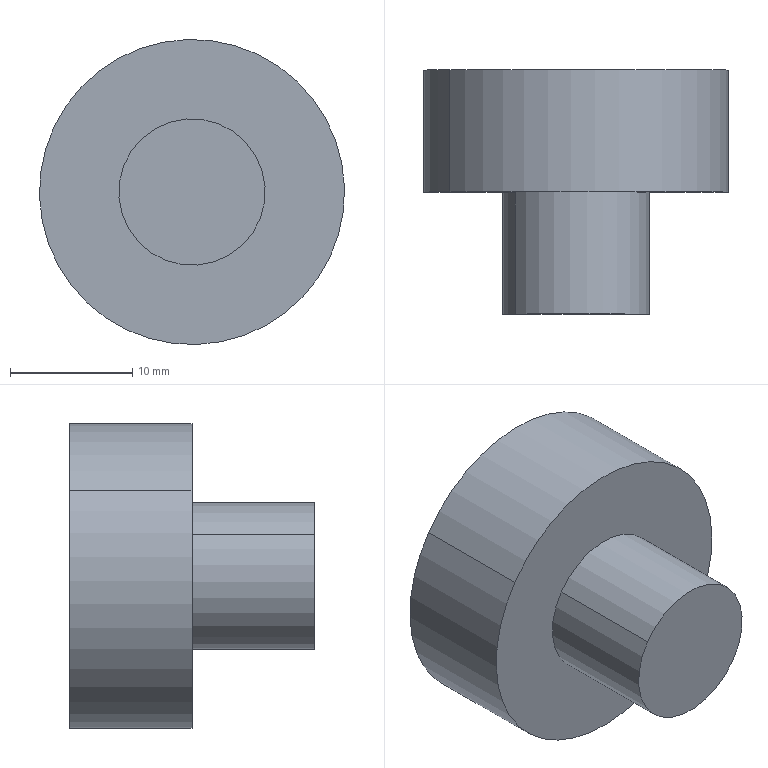Component | SolidWorks | UpperAxis-1_UpperSlideFixedBlock-1 | 1 solid | 10 faces | box 25 x 20 x 25 mm | volume 5870 mm3 | cylinder 6 | plane 4 | commonest cylinder face diameters 5.2 x2 12 x2 25 x2
build123d program:
from build123d import *

# Parameters (mm, degrees)
SKETCH1_R           = 12.5
BOSS_EXTRUDE1_DEPTH = 10
SKETCH2_R           = 6
BOSS_EXTRUDE2_DEPTH = 10
SKETCH3_R           = 2.6
CUT_EXTRUDE1_DEPTH  = 8


with BuildPart() as part:
    # Sketch1 → Boss-Extrude1 (new body)
    with BuildSketch(Plane.XY):
        Circle(SKETCH1_R)
    extrude(amount=BOSS_EXTRUDE1_DEPTH)

    # Sketch2 → Boss-Extrude2 (add)
    with BuildSketch(Plane.XY.offset(10)):
        Circle(SKETCH2_R)
    extrude(amount=BOSS_EXTRUDE2_DEPTH)

    # Sketch3 → Cut-Extrude1 (cut)
    with BuildSketch(Plane(origin=(0, 0, 0), x_dir=(-1, 0, 0), z_dir=(0, 0, -1))):
        Circle(SKETCH3_R)
    extrude(amount=-CUT_EXTRUDE1_DEPTH, mode=Mode.SUBTRACT)


solid = part.part

# Placed as in the assembly
solid = solid.moved(Location((-778.65, 394.568, -31.569), (90, 0, 0)))
STEP:
#1=COLOUR_RGB('',0.7922,0.8196,0.9333);
#2=FILL_AREA_STYLE_COLOUR('',#1);
#3=FILL_AREA_STYLE('',(#2));
#4=SURFACE_STYLE_FILL_AREA(#3);
#5=SURFACE_SIDE_STYLE('',(#4));
#6=SURFACE_STYLE_USAGE(.BOTH.,#5);
#7=PRESENTATION_STYLE_ASSIGNMENT((#6));
#8=CARTESIAN_POINT('',(-30.571,15.219,-1.301));
#9=VERTEX_POINT('',#8);
#10=CARTESIAN_POINT('',(-30.74,15.219,-1.185));
#11=VERTEX_POINT('',#10);
#12=CARTESIAN_POINT('',(-30.655,15.219,-1.243));
#13=DIRECTION('',(-0.,1.,0.));
#14=DIRECTION('',(-0.8265,0.,0.563));
#15=AXIS2_PLACEMENT_3D('',#12,#13,#14);
#16=CIRCLE('',#15,0.1024);
#17=EDGE_CURVE('',#9,#11,#16,.T.);
#18=ORIENTED_EDGE('',*,*,#17,.F.);
#19=CARTESIAN_POINT('',(-30.571,15.534,-1.301));
#20=VERTEX_POINT('',#19);
#21=CARTESIAN_POINT('',(-30.571,15.219,-1.301));
#22=DIRECTION('',(-0.,1.,0.));
#23=VECTOR('',#22,39.37);
#24=LINE('',#21,#23);
#25=EDGE_CURVE('',#9,#20,#24,.T.);
#26=ORIENTED_EDGE('',*,*,#25,.T.);
#27=CARTESIAN_POINT('',(-30.74,15.534,-1.185));
#28=VERTEX_POINT('',#27);
#29=CARTESIAN_POINT('',(-30.655,15.534,-1.243));
#30=DIRECTION('',(-0.,1.,0.));
#31=DIRECTION('',(-0.8265,0.,0.563));
#32=AXIS2_PLACEMENT_3D('',#29,#30,#31);
#33=CIRCLE('',#32,0.1024);
#34=EDGE_CURVE('',#20,#28,#33,.T.);
#35=ORIENTED_EDGE('',*,*,#34,.T.);
#36=CARTESIAN_POINT('',(-30.74,15.219,-1.185));
#37=DIRECTION('',(-0.,1.,0.));
#38=VECTOR('',#37,39.37);
#39=LINE('',#36,#38);
#40=EDGE_CURVE('',#11,#28,#39,.T.);
#41=ORIENTED_EDGE('',*,*,#40,.F.);
#42=EDGE_LOOP('',(#18,#26,#35,#41));
#43=FACE_OUTER_BOUND('',#42,.T.);
#44=CARTESIAN_POINT('',(-30.655,15.219,-1.243));
#45=DIRECTION('',(-0.,1.,0.));
#46=DIRECTION('',(-0.8265,0.,0.563));
#47=AXIS2_PLACEMENT_3D('',#44,#45,#46);
#48=CYLINDRICAL_SURFACE('',#47,0.1024);
#49=ADVANCED_FACE('',(#43),#48,.F.);
#50=CARTESIAN_POINT('',(-30.46,14.747,-1.376));
#51=VERTEX_POINT('',#50);
#52=CARTESIAN_POINT('',(-30.851,14.747,-1.11));
#53=VERTEX_POINT('',#52);
#54=CARTESIAN_POINT('',(-30.655,14.747,-1.243));
#55=DIRECTION('',(0.,-1.,-0.));
#56=DIRECTION('',(0.8265,0.,-0.563));
#57=AXIS2_PLACEMENT_3D('',#54,#55,#56);
#58=CIRCLE('',#57,0.2362);
#59=EDGE_CURVE('',#51,#53,#58,.T.);
#60=ORIENTED_EDGE('',*,*,#59,.F.);
#61=CARTESIAN_POINT('',(-30.46,15.14,-1.376));
#62=VERTEX_POINT('',#61);
#63=CARTESIAN_POINT('',(-30.46,14.747,-1.376));
#64=DIRECTION('',(-0.,1.,0.));
#65=VECTOR('',#64,39.37);
#66=LINE('',#63,#65);
#67=EDGE_CURVE('',#51,#62,#66,.T.);
#68=ORIENTED_EDGE('',*,*,#67,.T.);
#69=CARTESIAN_POINT('',(-30.851,15.14,-1.11));
#70=VERTEX_POINT('',#69);
#71=CARTESIAN_POINT('',(-30.655,15.14,-1.243));
#72=DIRECTION('',(0.,-1.,-0.));
#73=DIRECTION('',(0.8265,0.,-0.563));
#74=AXIS2_PLACEMENT_3D('',#71,#72,#73);
#75=CIRCLE('',#74,0.2362);
#76=EDGE_CURVE('',#62,#70,#75,.T.);
#77=ORIENTED_EDGE('',*,*,#76,.T.);
#78=CARTESIAN_POINT('',(-30.851,14.747,-1.11));
#79=DIRECTION('',(-0.,1.,0.));
#80=VECTOR('',#79,39.37);
#81=LINE('',#78,#80);
#82=EDGE_CURVE('',#53,#70,#81,.T.);
#83=ORIENTED_EDGE('',*,*,#82,.F.);
#84=EDGE_LOOP('',(#60,#68,#77,#83));
#85=FACE_OUTER_BOUND('',#84,.T.);
#86=CARTESIAN_POINT('',(-30.655,14.747,-1.243));
#87=DIRECTION('',(-0.,1.,0.));
#88=DIRECTION('',(-0.8265,0.,0.563));
#89=AXIS2_PLACEMENT_3D('',#86,#87,#88);
#90=CYLINDRICAL_SURFACE('',#89,0.2362);
#91=ADVANCED_FACE('',(#85),#90,.T.);
#92=CARTESIAN_POINT('',(-30.249,15.14,-1.52));
#93=VERTEX_POINT('',#92);
#94=CARTESIAN_POINT('',(-31.062,15.14,-0.9658));
#95=VERTEX_POINT('',#94);
#96=CARTESIAN_POINT('',(-30.655,15.14,-1.243));
#97=DIRECTION('',(0.,-1.,-0.));
#98=DIRECTION('',(0.8265,0.,-0.563));
#99=AXIS2_PLACEMENT_3D('',#96,#97,#98);
#100=CIRCLE('',#99,0.4921);
#101=EDGE_CURVE('',#93,#95,#100,.T.);
#102=ORIENTED_EDGE('',*,*,#101,.F.);
#103=CARTESIAN_POINT('',(-30.249,15.534,-1.52));
#104=VERTEX_POINT('',#103);
#105=CARTESIAN_POINT('',(-30.249,15.14,-1.52));
#106=DIRECTION('',(-0.,1.,0.));
#107=VECTOR('',#106,39.37);
#108=LINE('',#105,#107);
#109=EDGE_CURVE('',#93,#104,#108,.T.);
#110=ORIENTED_EDGE('',*,*,#109,.T.);
#111=CARTESIAN_POINT('',(-31.062,15.534,-0.9658));
#112=VERTEX_POINT('',#111);
#113=CARTESIAN_POINT('',(-30.655,15.534,-1.243));
#114=DIRECTION('',(0.,-1.,-0.));
#115=DIRECTION('',(0.8265,0.,-0.563));
#116=AXIS2_PLACEMENT_3D('',#113,#114,#115);
#117=CIRCLE('',#116,0.4921);
#118=EDGE_CURVE('',#104,#112,#117,.T.);
#119=ORIENTED_EDGE('',*,*,#118,.T.);
#120=CARTESIAN_POINT('',(-31.062,15.14,-0.9658));
#121=DIRECTION('',(-0.,1.,0.));
#122=VECTOR('',#121,39.37);
#123=LINE('',#120,#122);
#124=EDGE_CURVE('',#95,#112,#123,.T.);
#125=ORIENTED_EDGE('',*,*,#124,.F.);
#126=EDGE_LOOP('',(#102,#110,#119,#125));
#127=FACE_OUTER_BOUND('',#126,.T.);
#128=CARTESIAN_POINT('',(-30.655,15.14,-1.243));
#129=DIRECTION('',(-0.,1.,0.));
#130=DIRECTION('',(-0.8265,0.,0.563));
#131=AXIS2_PLACEMENT_3D('',#128,#129,#130);
#132=CYLINDRICAL_SURFACE('',#131,0.4921);
#133=ADVANCED_FACE('',(#127),#132,.T.);
#134=CARTESIAN_POINT('',(-30.655,15.14,-1.243));
#135=DIRECTION('',(0.,-1.,-0.));
#136=DIRECTION('',(0.8265,0.,-0.563));
#137=AXIS2_PLACEMENT_3D('',#134,#135,#136);
#138=CIRCLE('',#137,0.4921);
#139=EDGE_CURVE('',#95,#93,#138,.T.);
#140=ORIENTED_EDGE('',*,*,#139,.T.);
#141=ORIENTED_EDGE('',*,*,#101,.T.);
#142=EDGE_LOOP('',(#140,#141));
#143=FACE_OUTER_BOUND('',#142,.T.);
#144=CARTESIAN_POINT('',(-30.655,15.14,-1.243));
#145=DIRECTION('',(0.,-1.,-0.));
#146=DIRECTION('',(0.8265,0.,-0.563));
#147=AXIS2_PLACEMENT_3D('',#144,#145,#146);
#148=CIRCLE('',#147,0.2362);
#149=EDGE_CURVE('',#70,#62,#148,.T.);
#150=ORIENTED_EDGE('',*,*,#149,.F.);
#151=ORIENTED_EDGE('',*,*,#76,.F.);
#152=EDGE_LOOP('',(#150,#151));
#153=FACE_BOUND('',#152,.T.);
#154=CARTESIAN_POINT('',(-30.655,15.14,-1.243));
#155=DIRECTION('',(0.,-1.,-0.));
#156=DIRECTION('',(0.8265,0.,-0.563));
#157=AXIS2_PLACEMENT_3D('',#154,#155,#156);
#158=PLANE('',#157);
#159=ADVANCED_FACE('',(#143,#153),#158,.T.);
#160=ORIENTED_EDGE('',*,*,#109,.F.);
#161=ORIENTED_EDGE('',*,*,#139,.F.);
#162=ORIENTED_EDGE('',*,*,#124,.T.);
#163=CARTESIAN_POINT('',(-30.655,15.534,-1.243));
#164=DIRECTION('',(0.,-1.,-0.));
#165=DIRECTION('',(0.8265,0.,-0.563));
#166=AXIS2_PLACEMENT_3D('',#163,#164,#165);
#167=CIRCLE('',#166,0.4921);
#168=EDGE_CURVE('',#112,#104,#167,.T.);
#169=ORIENTED_EDGE('',*,*,#168,.T.);
#170=EDGE_LOOP('',(#160,#161,#162,#169));
#171=FACE_OUTER_BOUND('',#170,.T.);
#172=CARTESIAN_POINT('',(-30.655,15.14,-1.243));
#173=DIRECTION('',(-0.,1.,0.));
#174=DIRECTION('',(-0.8265,0.,0.563));
#175=AXIS2_PLACEMENT_3D('',#172,#173,#174);
#176=CYLINDRICAL_SURFACE('',#175,0.4921);
#177=ADVANCED_FACE('',(#171),#176,.T.);
#178=CARTESIAN_POINT('',(-30.655,15.534,-1.243));
#179=DIRECTION('',(-0.,1.,0.));
#180=DIRECTION('',(-0.8265,0.,0.563));
#181=AXIS2_PLACEMENT_3D('',#178,#179,#180);
#182=CIRCLE('',#181,0.1024);
#183=EDGE_CURVE('',#28,#20,#182,.T.);
#184=ORIENTED_EDGE('',*,*,#183,.F.);
#185=ORIENTED_EDGE('',*,*,#34,.F.);
#186=EDGE_LOOP('',(#184,#185));
#187=FACE_BOUND('',#186,.T.);
#188=ORIENTED_EDGE('',*,*,#168,.F.);
#189=ORIENTED_EDGE('',*,*,#118,.F.);
#190=EDGE_LOOP('',(#188,#189));
#191=FACE_OUTER_BOUND('',#190,.T.);
#192=CARTESIAN_POINT('',(-30.655,15.534,-1.243));
#193=DIRECTION('',(0.,-1.,-0.));
#194=DIRECTION('',(0.8265,0.,-0.563));
#195=AXIS2_PLACEMENT_3D('',#192,#193,#194);
#196=PLANE('',#195);
#197=ADVANCED_FACE('',(#187,#191),#196,.F.);
#198=ORIENTED_EDGE('',*,*,#67,.F.);
#199=CARTESIAN_POINT('',(-30.655,14.747,-1.243));
#200=DIRECTION('',(0.,-1.,-0.));
#201=DIRECTION('',(0.8265,0.,-0.563));
#202=AXIS2_PLACEMENT_3D('',#199,#200,#201);
#203=CIRCLE('',#202,0.2362);
#204=EDGE_CURVE('',#53,#51,#203,.T.);
#205=ORIENTED_EDGE('',*,*,#204,.F.);
#206=ORIENTED_EDGE('',*,*,#82,.T.);
#207=ORIENTED_EDGE('',*,*,#149,.T.);
#208=EDGE_LOOP('',(#198,#205,#206,#207));
#209=FACE_OUTER_BOUND('',#208,.T.);
#210=CARTESIAN_POINT('',(-30.655,14.747,-1.243));
#211=DIRECTION('',(-0.,1.,0.));
#212=DIRECTION('',(-0.8265,0.,0.563));
#213=AXIS2_PLACEMENT_3D('',#210,#211,#212);
#214=CYLINDRICAL_SURFACE('',#213,0.2362);
#215=ADVANCED_FACE('',(#209),#214,.T.);
#216=ORIENTED_EDGE('',*,*,#204,.T.);
#217=ORIENTED_EDGE('',*,*,#59,.T.);
#218=EDGE_LOOP('',(#216,#217));
#219=FACE_OUTER_BOUND('',#218,.T.);
#220=CARTESIAN_POINT('',(-30.655,14.747,-1.243));
#221=DIRECTION('',(0.,-1.,-0.));
#222=DIRECTION('',(0.8265,0.,-0.563));
#223=AXIS2_PLACEMENT_3D('',#220,#221,#222);
#224=PLANE('',#223);
#225=ADVANCED_FACE('',(#219),#224,.T.);
#226=ORIENTED_EDGE('',*,*,#25,.F.);
#227=CARTESIAN_POINT('',(-30.655,15.219,-1.243));
#228=DIRECTION('',(-0.,1.,0.));
#229=DIRECTION('',(-0.8265,0.,0.563));
#230=AXIS2_PLACEMENT_3D('',#227,#228,#229);
#231=CIRCLE('',#230,0.1024);
#232=EDGE_CURVE('',#11,#9,#231,.T.);
#233=ORIENTED_EDGE('',*,*,#232,.F.);
#234=ORIENTED_EDGE('',*,*,#40,.T.);
#235=ORIENTED_EDGE('',*,*,#183,.T.);
#236=EDGE_LOOP('',(#226,#233,#234,#235));
#237=FACE_OUTER_BOUND('',#236,.T.);
#238=CARTESIAN_POINT('',(-30.655,15.219,-1.243));
#239=DIRECTION('',(-0.,1.,0.));
#240=DIRECTION('',(-0.8265,0.,0.563));
#241=AXIS2_PLACEMENT_3D('',#238,#239,#240);
#242=CYLINDRICAL_SURFACE('',#241,0.1024);
#243=ADVANCED_FACE('',(#237),#242,.F.);
#244=ORIENTED_EDGE('',*,*,#232,.T.);
#245=ORIENTED_EDGE('',*,*,#17,.T.);
#246=EDGE_LOOP('',(#244,#245));
#247=FACE_OUTER_BOUND('',#246,.T.);
#248=CARTESIAN_POINT('',(-30.655,15.219,-1.243));
#249=DIRECTION('',(-0.,1.,0.));
#250=DIRECTION('',(-0.8265,-0.,0.563));
#251=AXIS2_PLACEMENT_3D('',#248,#249,#250);
#252=PLANE('',#251);
#253=ADVANCED_FACE('',(#247),#252,.T.);
#254=CLOSED_SHELL('',(#49,#91,#133,#159,#177,#197,#215,#225,#243,#253));
#255=MANIFOLD_SOLID_BREP('',#254);
#256=STYLED_ITEM('',(#7),#255);
#257=PRESENTATION_LAYER_ASSIGNMENT('','',(#256));
#258=CARTESIAN_POINT('',(0.,0.,0.));
#259=DIRECTION('',(0.,0.,1.));
#260=DIRECTION('',(1.,0.,0.));
#261=AXIS2_PLACEMENT_3D('',#258,#259,#260);
#262=(LENGTH_UNIT()NAMED_UNIT(*)SI_UNIT($,.METRE.));
#263=LENGTH_MEASURE_WITH_UNIT(LENGTH_MEASURE(0.0254),#262);
#264=DIMENSIONAL_EXPONENTS(1.,0.,0.,0.,0.,0.,0.);
#265=(CONVERSION_BASED_UNIT('',#263)LENGTH_UNIT()NAMED_UNIT(#264));
#266=UNCERTAINTY_MEASURE_WITH_UNIT(LENGTH_MEASURE(0.00001),#265,'','');
#267=(NAMED_UNIT(*)PLANE_ANGLE_UNIT()SI_UNIT($,.RADIAN.));
#268=(NAMED_UNIT(*)SI_UNIT($,.STERADIAN.)SOLID_ANGLE_UNIT());
#269=(GEOMETRIC_REPRESENTATION_CONTEXT(3)GLOBAL_UNCERTAINTY_ASSIGNED_CONTEXT((#266))GLOBAL_UNIT_ASSIGNED_CONTEXT((#265,#267,#268))REPRESENTATION_CONTEXT('',''));
#270=ADVANCED_BREP_SHAPE_REPRESENTATION('',(#255,#261),#269);
#271=(LENGTH_UNIT()NAMED_UNIT(*)SI_UNIT($,.METRE.));
#272=LENGTH_MEASURE_WITH_UNIT(LENGTH_MEASURE(0.0254),#271);
#273=DIMENSIONAL_EXPONENTS(1.,0.,0.,0.,0.,0.,0.);
#274=(CONVERSION_BASED_UNIT('',#272)LENGTH_UNIT()NAMED_UNIT(#273));
#275=UNCERTAINTY_MEASURE_WITH_UNIT(LENGTH_MEASURE(0.00001),#274,'','');
#276=(NAMED_UNIT(*)PLANE_ANGLE_UNIT()SI_UNIT($,.RADIAN.));
#277=(NAMED_UNIT(*)SI_UNIT($,.STERADIAN.)SOLID_ANGLE_UNIT());
#278=(GEOMETRIC_REPRESENTATION_CONTEXT(3)GLOBAL_UNCERTAINTY_ASSIGNED_CONTEXT((#275))GLOBAL_UNIT_ASSIGNED_CONTEXT((#274,#276,#277))REPRESENTATION_CONTEXT('',''));
#279=MECHANICAL_DESIGN_GEOMETRIC_PRESENTATION_REPRESENTATION('',(#256),#278);